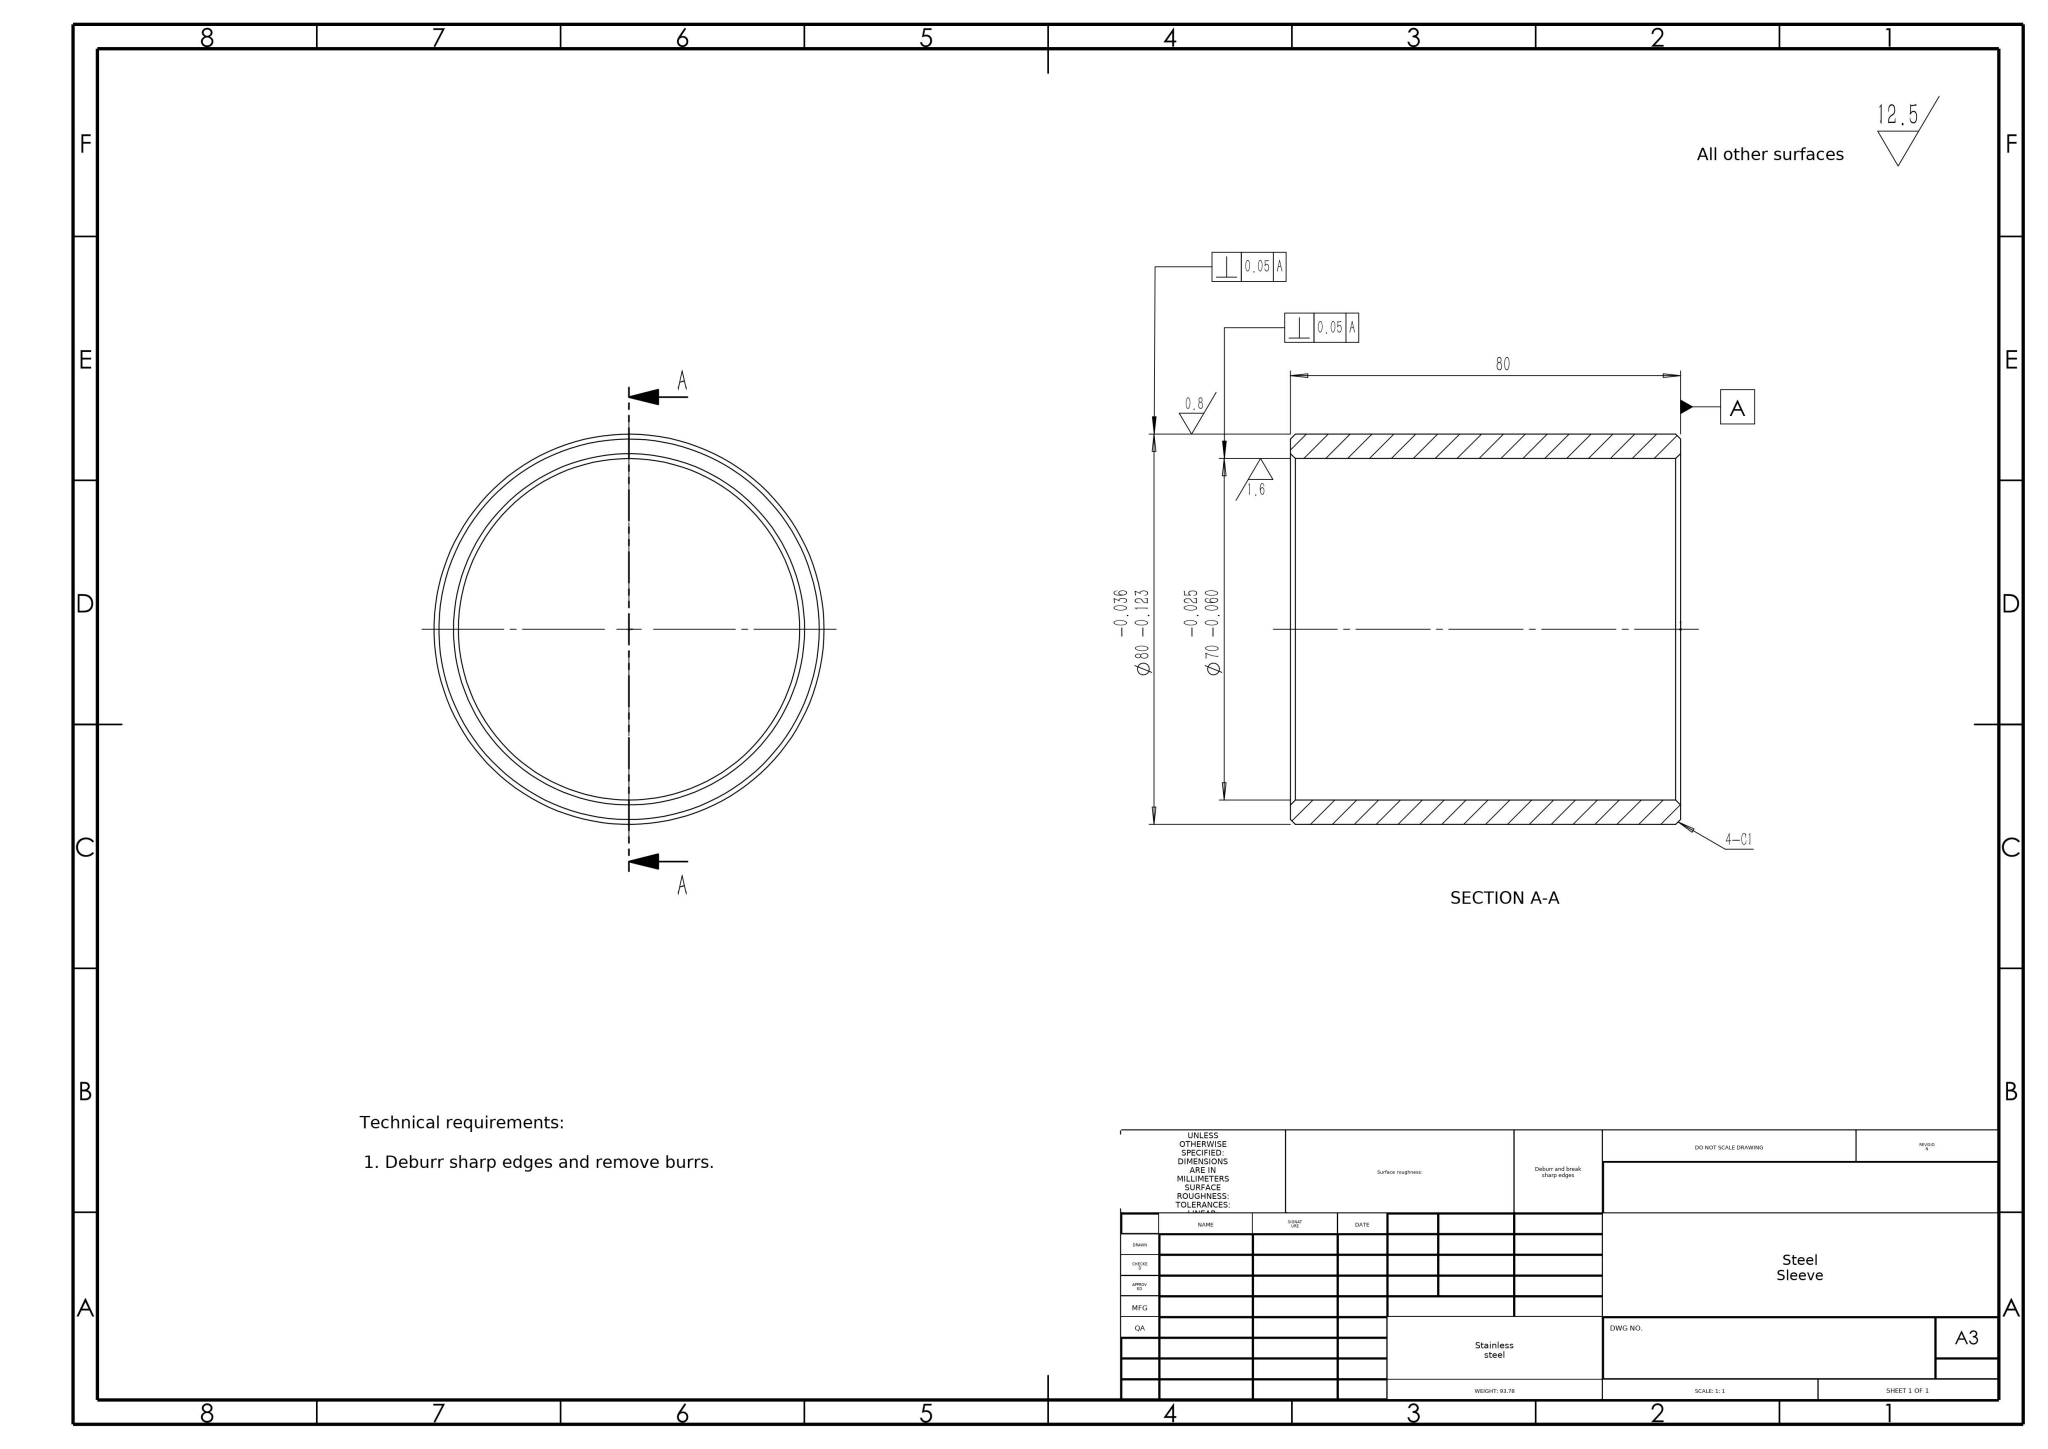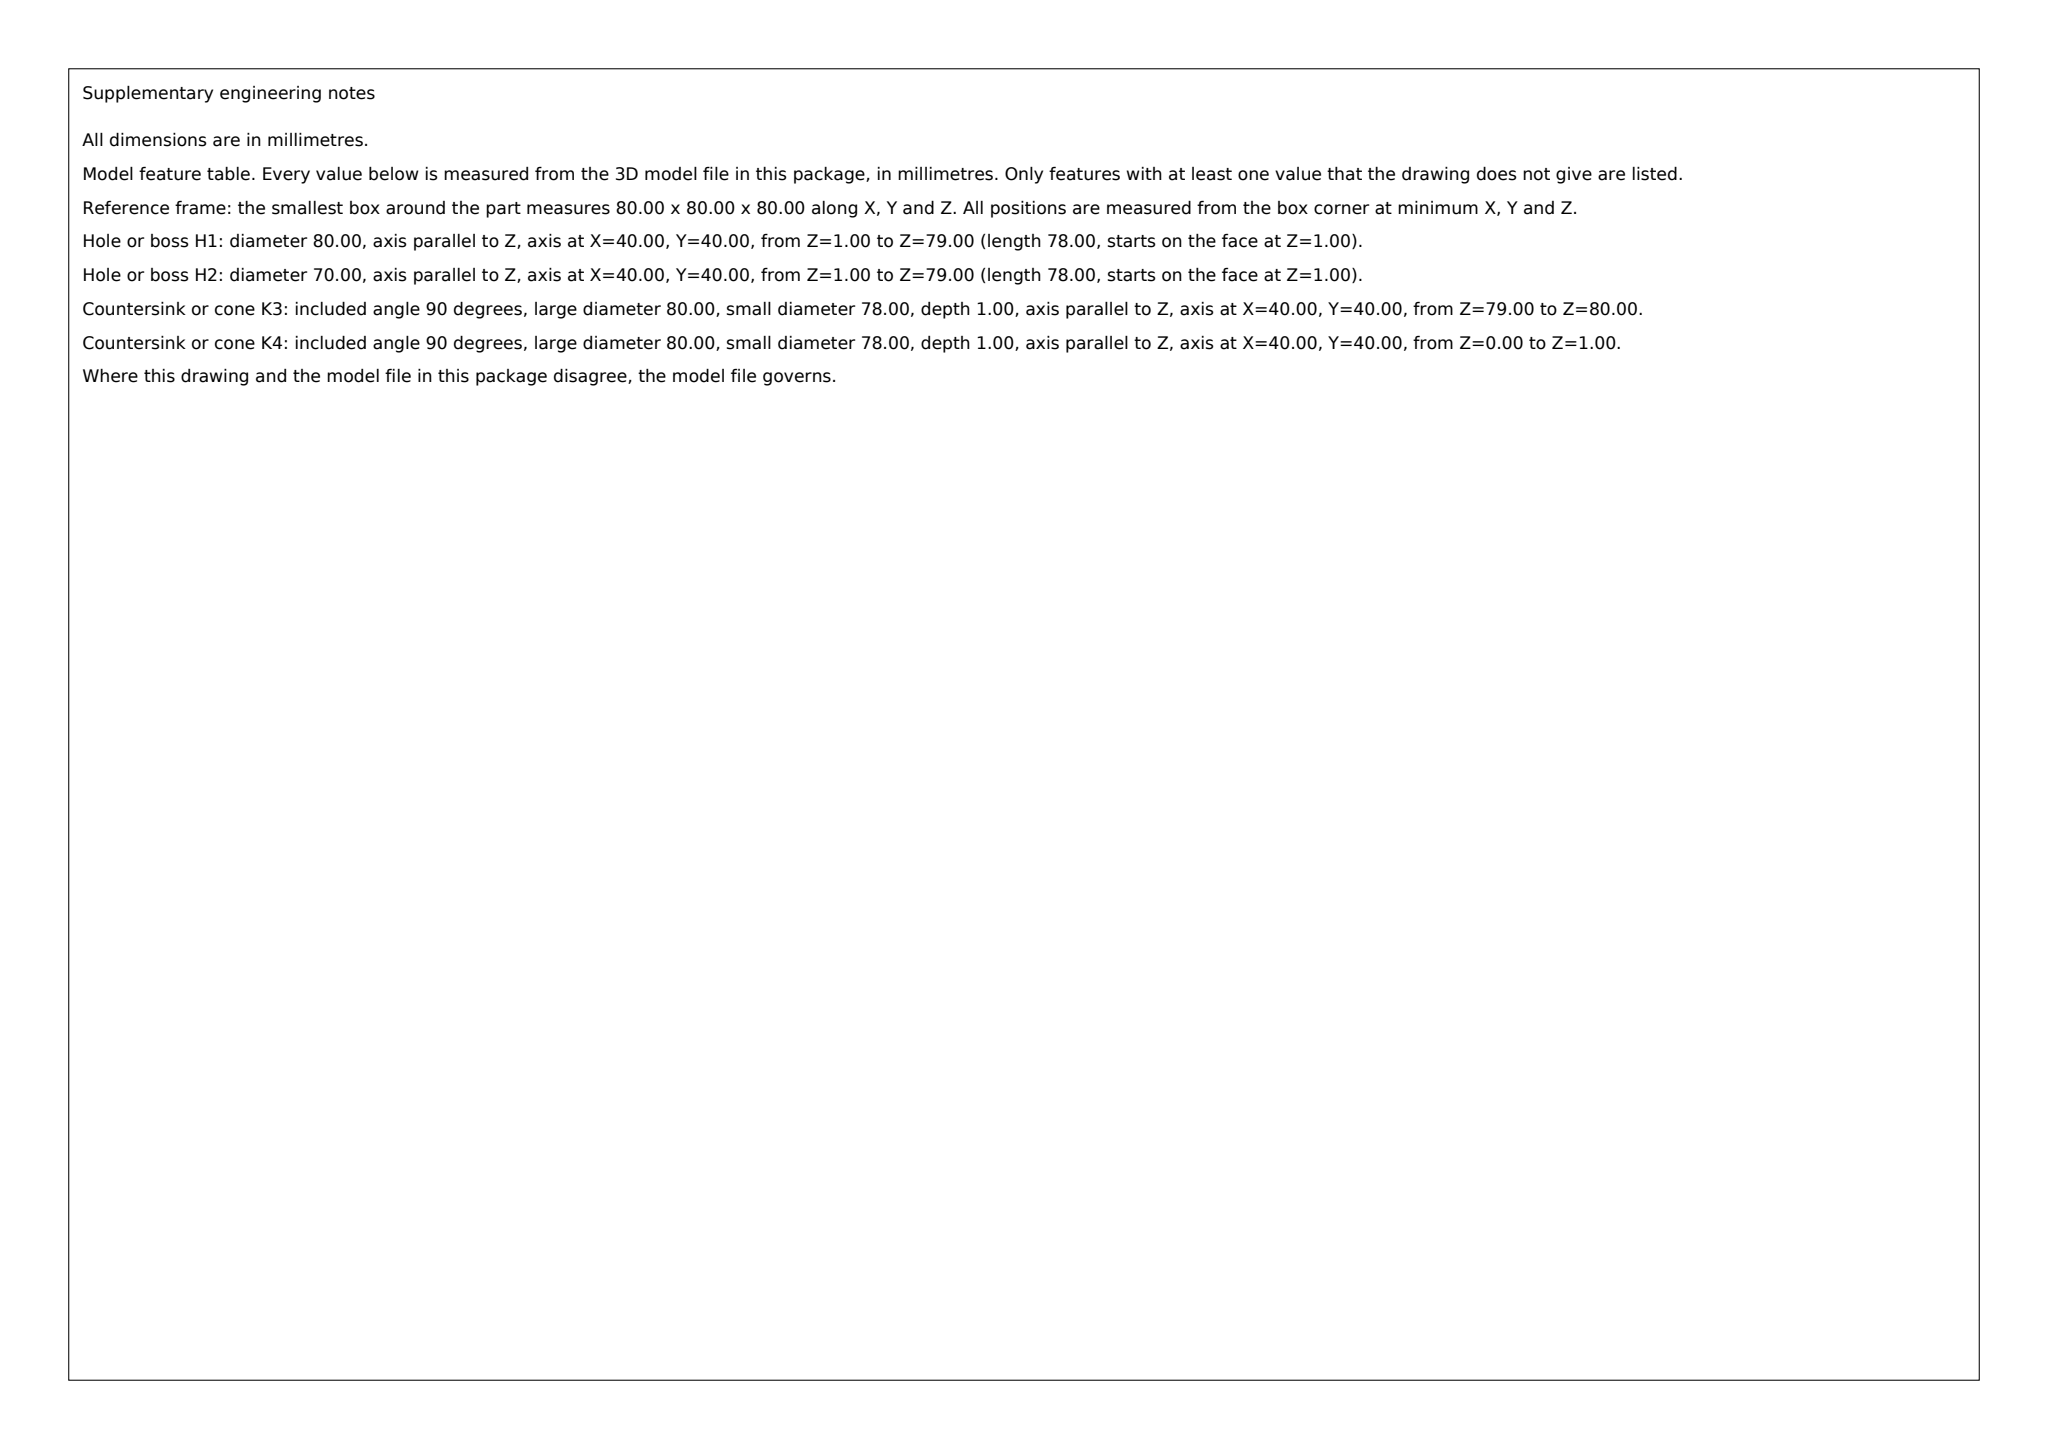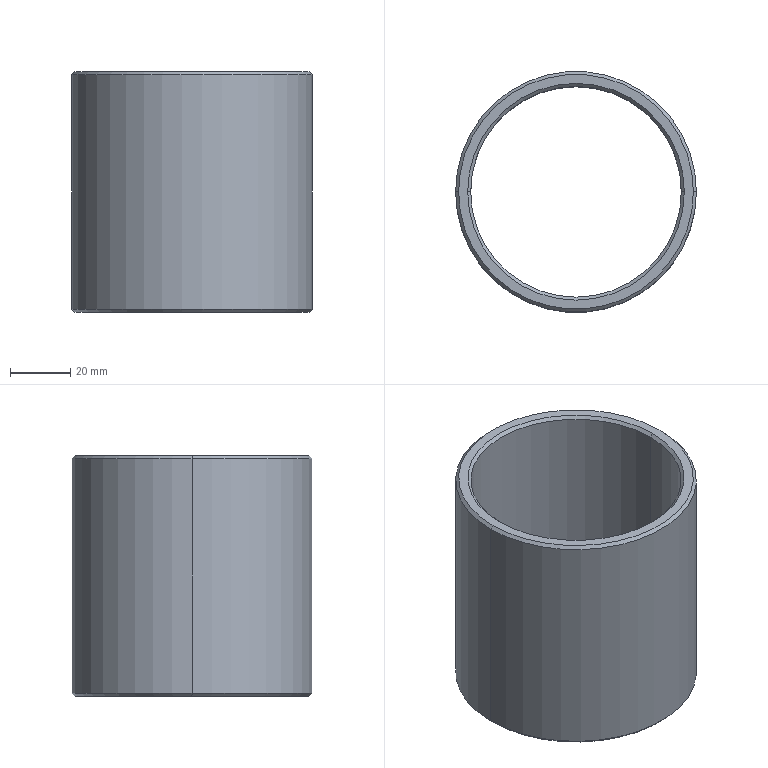Part | SolidWorks | mm | material Stainless steel | 1 solid | 14 faces | box 80 x 80 x 80 mm | volume 93777 mm3 | cone 8 | cylinder 4 | plane 2 | commonest cylinder face diameters 70 x2 80 x2
build123d program:
from build123d import *

# Parameters (mm, degrees)
SKETCH1_R           = 40
SKETCH1_R_2         = 35
BOSS_EXTRUDE1_DEPTH = 80
CHAMFER1_SIZE       = 1


with BuildPart() as part:
    # Sketch1 → Boss-Extrude1 (new body)
    with BuildSketch(Plane.XY):
        Circle(SKETCH1_R)
        Circle(SKETCH1_R_2, mode=Mode.SUBTRACT)
    extrude(amount=BOSS_EXTRUDE1_DEPTH)

    # Chamfer1
    chamfer1_edges = [part.edges().sort_by_distance(p)[0] for p in [
        (-40, 0, 0),
        (-40, 0, 80),
        (-35, 0, 0),
        (-35, 0, 80),
    ]]
    chamfer(chamfer1_edges, length=CHAMFER1_SIZE)


solid = part.part
STEP:
#1=CARTESIAN_POINT('',(-35.,0.,79.));
#2=VERTEX_POINT('',#1);
#3=CARTESIAN_POINT('',(35.,0.,79.));
#4=VERTEX_POINT('',#3);
#5=CARTESIAN_POINT('',(0.,0.,79.));
#6=DIRECTION('',(0.,0.,1.));
#7=DIRECTION('',(1.,0.,0.));
#8=AXIS2_PLACEMENT_3D('',#5,#6,#7);
#9=CIRCLE('',#8,35.);
#10=EDGE_CURVE('',#2,#4,#9,.T.);
#11=ORIENTED_EDGE('',*,*,#10,.F.);
#12=CARTESIAN_POINT('',(-36.,0.,80.));
#13=VERTEX_POINT('',#12);
#14=CARTESIAN_POINT('',(-35.,0.,79.));
#15=DIRECTION('',(-0.7071,0.,0.7071));
#16=VECTOR('',#15,1000.);
#17=LINE('',#14,#16);
#18=EDGE_CURVE('',#2,#13,#17,.T.);
#19=ORIENTED_EDGE('',*,*,#18,.T.);
#20=CARTESIAN_POINT('',(36.,0.,80.));
#21=VERTEX_POINT('',#20);
#22=CARTESIAN_POINT('',(0.,0.,80.));
#23=DIRECTION('',(0.,0.,-1.));
#24=DIRECTION('',(1.,0.,0.));
#25=AXIS2_PLACEMENT_3D('',#22,#23,#24);
#26=CIRCLE('',#25,36.);
#27=EDGE_CURVE('',#21,#13,#26,.T.);
#28=ORIENTED_EDGE('',*,*,#27,.F.);
#29=CARTESIAN_POINT('',(35.,0.,79.));
#30=DIRECTION('',(0.7071,0.,0.7071));
#31=VECTOR('',#30,1000.);
#32=LINE('',#29,#31);
#33=EDGE_CURVE('',#4,#21,#32,.T.);
#34=ORIENTED_EDGE('',*,*,#33,.F.);
#35=EDGE_LOOP('',(#11,#19,#28,#34));
#36=FACE_OUTER_BOUND('',#35,.T.);
#37=CARTESIAN_POINT('',(0.,0.,79.));
#38=DIRECTION('',(0.,0.,1.));
#39=DIRECTION('',(1.,0.,0.));
#40=AXIS2_PLACEMENT_3D('',#37,#38,#39);
#41=CONICAL_SURFACE('',#40,35.,0.7854);
#42=ADVANCED_FACE('',(#36),#41,.F.);
#43=CARTESIAN_POINT('',(39.,0.,80.));
#44=VERTEX_POINT('',#43);
#45=CARTESIAN_POINT('',(-39.,0.,80.));
#46=VERTEX_POINT('',#45);
#47=CARTESIAN_POINT('',(0.,0.,80.));
#48=DIRECTION('',(0.,0.,1.));
#49=DIRECTION('',(1.,0.,0.));
#50=AXIS2_PLACEMENT_3D('',#47,#48,#49);
#51=CIRCLE('',#50,39.);
#52=EDGE_CURVE('',#44,#46,#51,.T.);
#53=ORIENTED_EDGE('',*,*,#52,.F.);
#54=CARTESIAN_POINT('',(40.,0.,79.));
#55=VERTEX_POINT('',#54);
#56=CARTESIAN_POINT('',(39.,0.,80.));
#57=DIRECTION('',(0.7071,0.,-0.7071));
#58=VECTOR('',#57,1000.);
#59=LINE('',#56,#58);
#60=EDGE_CURVE('',#44,#55,#59,.T.);
#61=ORIENTED_EDGE('',*,*,#60,.T.);
#62=CARTESIAN_POINT('',(-40.,0.,79.));
#63=VERTEX_POINT('',#62);
#64=CARTESIAN_POINT('',(0.,0.,79.));
#65=DIRECTION('',(0.,0.,-1.));
#66=DIRECTION('',(1.,0.,0.));
#67=AXIS2_PLACEMENT_3D('',#64,#65,#66);
#68=CIRCLE('',#67,40.);
#69=EDGE_CURVE('',#63,#55,#68,.T.);
#70=ORIENTED_EDGE('',*,*,#69,.F.);
#71=CARTESIAN_POINT('',(-39.,0.,80.));
#72=DIRECTION('',(-0.7071,0.,-0.7071));
#73=VECTOR('',#72,1000.);
#74=LINE('',#71,#73);
#75=EDGE_CURVE('',#46,#63,#74,.T.);
#76=ORIENTED_EDGE('',*,*,#75,.F.);
#77=EDGE_LOOP('',(#53,#61,#70,#76));
#78=FACE_OUTER_BOUND('',#77,.T.);
#79=CARTESIAN_POINT('',(0.,0.,80.));
#80=DIRECTION('',(0.,0.,-1.));
#81=DIRECTION('',(-1.,0.,0.));
#82=AXIS2_PLACEMENT_3D('',#79,#80,#81);
#83=CONICAL_SURFACE('',#82,39.,0.7854);
#84=ADVANCED_FACE('',(#78),#83,.T.);
#85=CARTESIAN_POINT('',(-39.,0.,0.));
#86=VERTEX_POINT('',#85);
#87=CARTESIAN_POINT('',(39.,0.,0.));
#88=VERTEX_POINT('',#87);
#89=CARTESIAN_POINT('',(0.,0.,0.));
#90=DIRECTION('',(0.,0.,-1.));
#91=DIRECTION('',(1.,0.,0.));
#92=AXIS2_PLACEMENT_3D('',#89,#90,#91);
#93=CIRCLE('',#92,39.);
#94=EDGE_CURVE('',#86,#88,#93,.T.);
#95=ORIENTED_EDGE('',*,*,#94,.F.);
#96=CARTESIAN_POINT('',(-40.,0.,1.));
#97=VERTEX_POINT('',#96);
#98=CARTESIAN_POINT('',(-40.,0.,1.));
#99=DIRECTION('',(-0.7071,0.,0.7071));
#100=VECTOR('',#99,1000.);
#101=LINE('',#98,#100);
#102=EDGE_CURVE('',#86,#97,#101,.T.);
#103=ORIENTED_EDGE('',*,*,#102,.T.);
#104=CARTESIAN_POINT('',(40.,0.,1.));
#105=VERTEX_POINT('',#104);
#106=CARTESIAN_POINT('',(0.,0.,1.));
#107=DIRECTION('',(0.,0.,1.));
#108=DIRECTION('',(1.,0.,0.));
#109=AXIS2_PLACEMENT_3D('',#106,#107,#108);
#110=CIRCLE('',#109,40.);
#111=EDGE_CURVE('',#105,#97,#110,.T.);
#112=ORIENTED_EDGE('',*,*,#111,.F.);
#113=CARTESIAN_POINT('',(40.,0.,1.));
#114=DIRECTION('',(0.7071,0.,0.7071));
#115=VECTOR('',#114,1000.);
#116=LINE('',#113,#115);
#117=EDGE_CURVE('',#88,#105,#116,.T.);
#118=ORIENTED_EDGE('',*,*,#117,.F.);
#119=EDGE_LOOP('',(#95,#103,#112,#118));
#120=FACE_OUTER_BOUND('',#119,.T.);
#121=CARTESIAN_POINT('',(0.,0.,1.));
#122=DIRECTION('',(0.,0.,1.));
#123=DIRECTION('',(1.,0.,0.));
#124=AXIS2_PLACEMENT_3D('',#121,#122,#123);
#125=CONICAL_SURFACE('',#124,40.,0.7854);
#126=ADVANCED_FACE('',(#120),#125,.T.);
#127=CARTESIAN_POINT('',(35.,0.,1.));
#128=VERTEX_POINT('',#127);
#129=CARTESIAN_POINT('',(-35.,0.,1.));
#130=VERTEX_POINT('',#129);
#131=CARTESIAN_POINT('',(0.,0.,1.));
#132=DIRECTION('',(0.,0.,-1.));
#133=DIRECTION('',(1.,0.,0.));
#134=AXIS2_PLACEMENT_3D('',#131,#132,#133);
#135=CIRCLE('',#134,35.);
#136=EDGE_CURVE('',#128,#130,#135,.T.);
#137=ORIENTED_EDGE('',*,*,#136,.F.);
#138=CARTESIAN_POINT('',(36.,0.,0.));
#139=VERTEX_POINT('',#138);
#140=CARTESIAN_POINT('',(36.,0.,0.));
#141=DIRECTION('',(0.7071,0.,-0.7071));
#142=VECTOR('',#141,1000.);
#143=LINE('',#140,#142);
#144=EDGE_CURVE('',#128,#139,#143,.T.);
#145=ORIENTED_EDGE('',*,*,#144,.T.);
#146=CARTESIAN_POINT('',(-36.,0.,0.));
#147=VERTEX_POINT('',#146);
#148=CARTESIAN_POINT('',(0.,0.,0.));
#149=DIRECTION('',(0.,0.,1.));
#150=DIRECTION('',(1.,0.,0.));
#151=AXIS2_PLACEMENT_3D('',#148,#149,#150);
#152=CIRCLE('',#151,36.);
#153=EDGE_CURVE('',#147,#139,#152,.T.);
#154=ORIENTED_EDGE('',*,*,#153,.F.);
#155=CARTESIAN_POINT('',(-36.,0.,0.));
#156=DIRECTION('',(-0.7071,0.,-0.7071));
#157=VECTOR('',#156,1000.);
#158=LINE('',#155,#157);
#159=EDGE_CURVE('',#130,#147,#158,.T.);
#160=ORIENTED_EDGE('',*,*,#159,.F.);
#161=EDGE_LOOP('',(#137,#145,#154,#160));
#162=FACE_OUTER_BOUND('',#161,.T.);
#163=CARTESIAN_POINT('',(0.,0.,0.));
#164=DIRECTION('',(0.,0.,-1.));
#165=DIRECTION('',(-1.,0.,0.));
#166=AXIS2_PLACEMENT_3D('',#163,#164,#165);
#167=CONICAL_SURFACE('',#166,36.,0.7854);
#168=ADVANCED_FACE('',(#162),#167,.F.);
#169=ORIENTED_EDGE('',*,*,#10,.T.);
#170=CARTESIAN_POINT('',(35.,0.,80.));
#171=DIRECTION('',(0.,0.,-1.));
#172=VECTOR('',#171,1000.);
#173=LINE('',#170,#172);
#174=EDGE_CURVE('',#4,#128,#173,.T.);
#175=ORIENTED_EDGE('',*,*,#174,.T.);
#176=ORIENTED_EDGE('',*,*,#136,.T.);
#177=CARTESIAN_POINT('',(-35.,0.,80.));
#178=DIRECTION('',(0.,0.,-1.));
#179=VECTOR('',#178,1000.);
#180=LINE('',#177,#179);
#181=EDGE_CURVE('',#2,#130,#180,.T.);
#182=ORIENTED_EDGE('',*,*,#181,.F.);
#183=EDGE_LOOP('',(#169,#175,#176,#182));
#184=FACE_OUTER_BOUND('',#183,.T.);
#185=CARTESIAN_POINT('',(0.,0.,80.));
#186=DIRECTION('',(0.,0.,-1.));
#187=DIRECTION('',(-1.,0.,0.));
#188=AXIS2_PLACEMENT_3D('',#185,#186,#187);
#189=CYLINDRICAL_SURFACE('',#188,35.);
#190=ADVANCED_FACE('',(#184),#189,.F.);
#191=ORIENTED_EDGE('',*,*,#69,.T.);
#192=CARTESIAN_POINT('',(40.,0.,80.));
#193=DIRECTION('',(0.,0.,-1.));
#194=VECTOR('',#193,1000.);
#195=LINE('',#192,#194);
#196=EDGE_CURVE('',#55,#105,#195,.T.);
#197=ORIENTED_EDGE('',*,*,#196,.T.);
#198=ORIENTED_EDGE('',*,*,#111,.T.);
#199=CARTESIAN_POINT('',(-40.,0.,80.));
#200=DIRECTION('',(0.,0.,-1.));
#201=VECTOR('',#200,1000.);
#202=LINE('',#199,#201);
#203=EDGE_CURVE('',#63,#97,#202,.T.);
#204=ORIENTED_EDGE('',*,*,#203,.F.);
#205=EDGE_LOOP('',(#191,#197,#198,#204));
#206=FACE_OUTER_BOUND('',#205,.T.);
#207=CARTESIAN_POINT('',(0.,0.,80.));
#208=DIRECTION('',(0.,0.,-1.));
#209=DIRECTION('',(-1.,0.,0.));
#210=AXIS2_PLACEMENT_3D('',#207,#208,#209);
#211=CYLINDRICAL_SURFACE('',#210,40.);
#212=ADVANCED_FACE('',(#206),#211,.T.);
#213=CARTESIAN_POINT('',(0.,0.,80.));
#214=DIRECTION('',(0.,0.,1.));
#215=DIRECTION('',(1.,0.,0.));
#216=AXIS2_PLACEMENT_3D('',#213,#214,#215);
#217=CIRCLE('',#216,39.);
#218=EDGE_CURVE('',#46,#44,#217,.T.);
#219=ORIENTED_EDGE('',*,*,#218,.T.);
#220=ORIENTED_EDGE('',*,*,#52,.T.);
#221=EDGE_LOOP('',(#219,#220));
#222=FACE_OUTER_BOUND('',#221,.T.);
#223=ORIENTED_EDGE('',*,*,#27,.T.);
#224=CARTESIAN_POINT('',(0.,0.,80.));
#225=DIRECTION('',(0.,0.,-1.));
#226=DIRECTION('',(1.,0.,0.));
#227=AXIS2_PLACEMENT_3D('',#224,#225,#226);
#228=CIRCLE('',#227,36.);
#229=EDGE_CURVE('',#13,#21,#228,.T.);
#230=ORIENTED_EDGE('',*,*,#229,.T.);
#231=EDGE_LOOP('',(#223,#230));
#232=FACE_BOUND('',#231,.T.);
#233=CARTESIAN_POINT('',(0.,0.,80.));
#234=DIRECTION('',(0.,0.,1.));
#235=DIRECTION('',(1.,0.,0.));
#236=AXIS2_PLACEMENT_3D('',#233,#234,#235);
#237=PLANE('',#236);
#238=ADVANCED_FACE('',(#222,#232),#237,.T.);
#239=ORIENTED_EDGE('',*,*,#153,.T.);
#240=CARTESIAN_POINT('',(0.,0.,0.));
#241=DIRECTION('',(0.,0.,1.));
#242=DIRECTION('',(1.,0.,0.));
#243=AXIS2_PLACEMENT_3D('',#240,#241,#242);
#244=CIRCLE('',#243,36.);
#245=EDGE_CURVE('',#139,#147,#244,.T.);
#246=ORIENTED_EDGE('',*,*,#245,.T.);
#247=EDGE_LOOP('',(#239,#246));
#248=FACE_BOUND('',#247,.T.);
#249=CARTESIAN_POINT('',(0.,0.,0.));
#250=DIRECTION('',(0.,0.,-1.));
#251=DIRECTION('',(1.,0.,0.));
#252=AXIS2_PLACEMENT_3D('',#249,#250,#251);
#253=CIRCLE('',#252,39.);
#254=EDGE_CURVE('',#88,#86,#253,.T.);
#255=ORIENTED_EDGE('',*,*,#254,.T.);
#256=ORIENTED_EDGE('',*,*,#94,.T.);
#257=EDGE_LOOP('',(#255,#256));
#258=FACE_OUTER_BOUND('',#257,.T.);
#259=CARTESIAN_POINT('',(0.,0.,0.));
#260=DIRECTION('',(0.,0.,1.));
#261=DIRECTION('',(1.,0.,0.));
#262=AXIS2_PLACEMENT_3D('',#259,#260,#261);
#263=PLANE('',#262);
#264=ADVANCED_FACE('',(#248,#258),#263,.F.);
#265=ORIENTED_EDGE('',*,*,#196,.F.);
#266=CARTESIAN_POINT('',(0.,0.,79.));
#267=DIRECTION('',(0.,0.,-1.));
#268=DIRECTION('',(1.,0.,0.));
#269=AXIS2_PLACEMENT_3D('',#266,#267,#268);
#270=CIRCLE('',#269,40.);
#271=EDGE_CURVE('',#55,#63,#270,.T.);
#272=ORIENTED_EDGE('',*,*,#271,.T.);
#273=ORIENTED_EDGE('',*,*,#203,.T.);
#274=CARTESIAN_POINT('',(0.,0.,1.));
#275=DIRECTION('',(0.,0.,1.));
#276=DIRECTION('',(1.,0.,0.));
#277=AXIS2_PLACEMENT_3D('',#274,#275,#276);
#278=CIRCLE('',#277,40.);
#279=EDGE_CURVE('',#97,#105,#278,.T.);
#280=ORIENTED_EDGE('',*,*,#279,.T.);
#281=EDGE_LOOP('',(#265,#272,#273,#280));
#282=FACE_OUTER_BOUND('',#281,.T.);
#283=CARTESIAN_POINT('',(0.,0.,80.));
#284=DIRECTION('',(0.,0.,-1.));
#285=DIRECTION('',(-1.,0.,0.));
#286=AXIS2_PLACEMENT_3D('',#283,#284,#285);
#287=CYLINDRICAL_SURFACE('',#286,40.);
#288=ADVANCED_FACE('',(#282),#287,.T.);
#289=ORIENTED_EDGE('',*,*,#174,.F.);
#290=CARTESIAN_POINT('',(0.,0.,79.));
#291=DIRECTION('',(0.,0.,1.));
#292=DIRECTION('',(1.,0.,0.));
#293=AXIS2_PLACEMENT_3D('',#290,#291,#292);
#294=CIRCLE('',#293,35.);
#295=EDGE_CURVE('',#4,#2,#294,.T.);
#296=ORIENTED_EDGE('',*,*,#295,.T.);
#297=ORIENTED_EDGE('',*,*,#181,.T.);
#298=CARTESIAN_POINT('',(0.,0.,1.));
#299=DIRECTION('',(0.,0.,-1.));
#300=DIRECTION('',(1.,0.,0.));
#301=AXIS2_PLACEMENT_3D('',#298,#299,#300);
#302=CIRCLE('',#301,35.);
#303=EDGE_CURVE('',#130,#128,#302,.T.);
#304=ORIENTED_EDGE('',*,*,#303,.T.);
#305=EDGE_LOOP('',(#289,#296,#297,#304));
#306=FACE_OUTER_BOUND('',#305,.T.);
#307=CARTESIAN_POINT('',(0.,0.,80.));
#308=DIRECTION('',(0.,0.,-1.));
#309=DIRECTION('',(-1.,0.,0.));
#310=AXIS2_PLACEMENT_3D('',#307,#308,#309);
#311=CYLINDRICAL_SURFACE('',#310,35.);
#312=ADVANCED_FACE('',(#306),#311,.F.);
#313=ORIENTED_EDGE('',*,*,#144,.F.);
#314=ORIENTED_EDGE('',*,*,#303,.F.);
#315=ORIENTED_EDGE('',*,*,#159,.T.);
#316=ORIENTED_EDGE('',*,*,#245,.F.);
#317=EDGE_LOOP('',(#313,#314,#315,#316));
#318=FACE_OUTER_BOUND('',#317,.T.);
#319=CARTESIAN_POINT('',(0.,0.,0.));
#320=DIRECTION('',(0.,0.,-1.));
#321=DIRECTION('',(-1.,0.,0.));
#322=AXIS2_PLACEMENT_3D('',#319,#320,#321);
#323=CONICAL_SURFACE('',#322,36.,0.7854);
#324=ADVANCED_FACE('',(#318),#323,.F.);
#325=ORIENTED_EDGE('',*,*,#102,.F.);
#326=ORIENTED_EDGE('',*,*,#254,.F.);
#327=ORIENTED_EDGE('',*,*,#117,.T.);
#328=ORIENTED_EDGE('',*,*,#279,.F.);
#329=EDGE_LOOP('',(#325,#326,#327,#328));
#330=FACE_OUTER_BOUND('',#329,.T.);
#331=CARTESIAN_POINT('',(0.,0.,1.));
#332=DIRECTION('',(0.,0.,1.));
#333=DIRECTION('',(1.,0.,0.));
#334=AXIS2_PLACEMENT_3D('',#331,#332,#333);
#335=CONICAL_SURFACE('',#334,40.,0.7854);
#336=ADVANCED_FACE('',(#330),#335,.T.);
#337=ORIENTED_EDGE('',*,*,#60,.F.);
#338=ORIENTED_EDGE('',*,*,#218,.F.);
#339=ORIENTED_EDGE('',*,*,#75,.T.);
#340=ORIENTED_EDGE('',*,*,#271,.F.);
#341=EDGE_LOOP('',(#337,#338,#339,#340));
#342=FACE_OUTER_BOUND('',#341,.T.);
#343=CARTESIAN_POINT('',(0.,0.,80.));
#344=DIRECTION('',(0.,0.,-1.));
#345=DIRECTION('',(-1.,0.,0.));
#346=AXIS2_PLACEMENT_3D('',#343,#344,#345);
#347=CONICAL_SURFACE('',#346,39.,0.7854);
#348=ADVANCED_FACE('',(#342),#347,.T.);
#349=ORIENTED_EDGE('',*,*,#18,.F.);
#350=ORIENTED_EDGE('',*,*,#295,.F.);
#351=ORIENTED_EDGE('',*,*,#33,.T.);
#352=ORIENTED_EDGE('',*,*,#229,.F.);
#353=EDGE_LOOP('',(#349,#350,#351,#352));
#354=FACE_OUTER_BOUND('',#353,.T.);
#355=CARTESIAN_POINT('',(0.,0.,79.));
#356=DIRECTION('',(0.,0.,1.));
#357=DIRECTION('',(1.,0.,0.));
#358=AXIS2_PLACEMENT_3D('',#355,#356,#357);
#359=CONICAL_SURFACE('',#358,35.,0.7854);
#360=ADVANCED_FACE('',(#354),#359,.F.);
#361=CLOSED_SHELL('',(#42,#84,#126,#168,#190,#212,#238,#264,#288,#312,#324,#336,#348,#360));
#362=MANIFOLD_SOLID_BREP('',#361);
#363=CARTESIAN_POINT('',(0.,0.,0.));
#364=DIRECTION('',(0.,0.,1.));
#365=DIRECTION('',(1.,0.,0.));
#366=AXIS2_PLACEMENT_3D('',#363,#364,#365);
#367=(LENGTH_UNIT()NAMED_UNIT(*)SI_UNIT(.MILLI.,.METRE.));
#368=UNCERTAINTY_MEASURE_WITH_UNIT(LENGTH_MEASURE(0.00001),#367,'','');
#369=(NAMED_UNIT(*)PLANE_ANGLE_UNIT()SI_UNIT($,.RADIAN.));
#370=(NAMED_UNIT(*)SI_UNIT($,.STERADIAN.)SOLID_ANGLE_UNIT());
#371=(GEOMETRIC_REPRESENTATION_CONTEXT(3)GLOBAL_UNCERTAINTY_ASSIGNED_CONTEXT((#368))GLOBAL_UNIT_ASSIGNED_CONTEXT((#367,#369,#370))REPRESENTATION_CONTEXT('',''));
#372=ADVANCED_BREP_SHAPE_REPRESENTATION('',(#362,#366),#371);